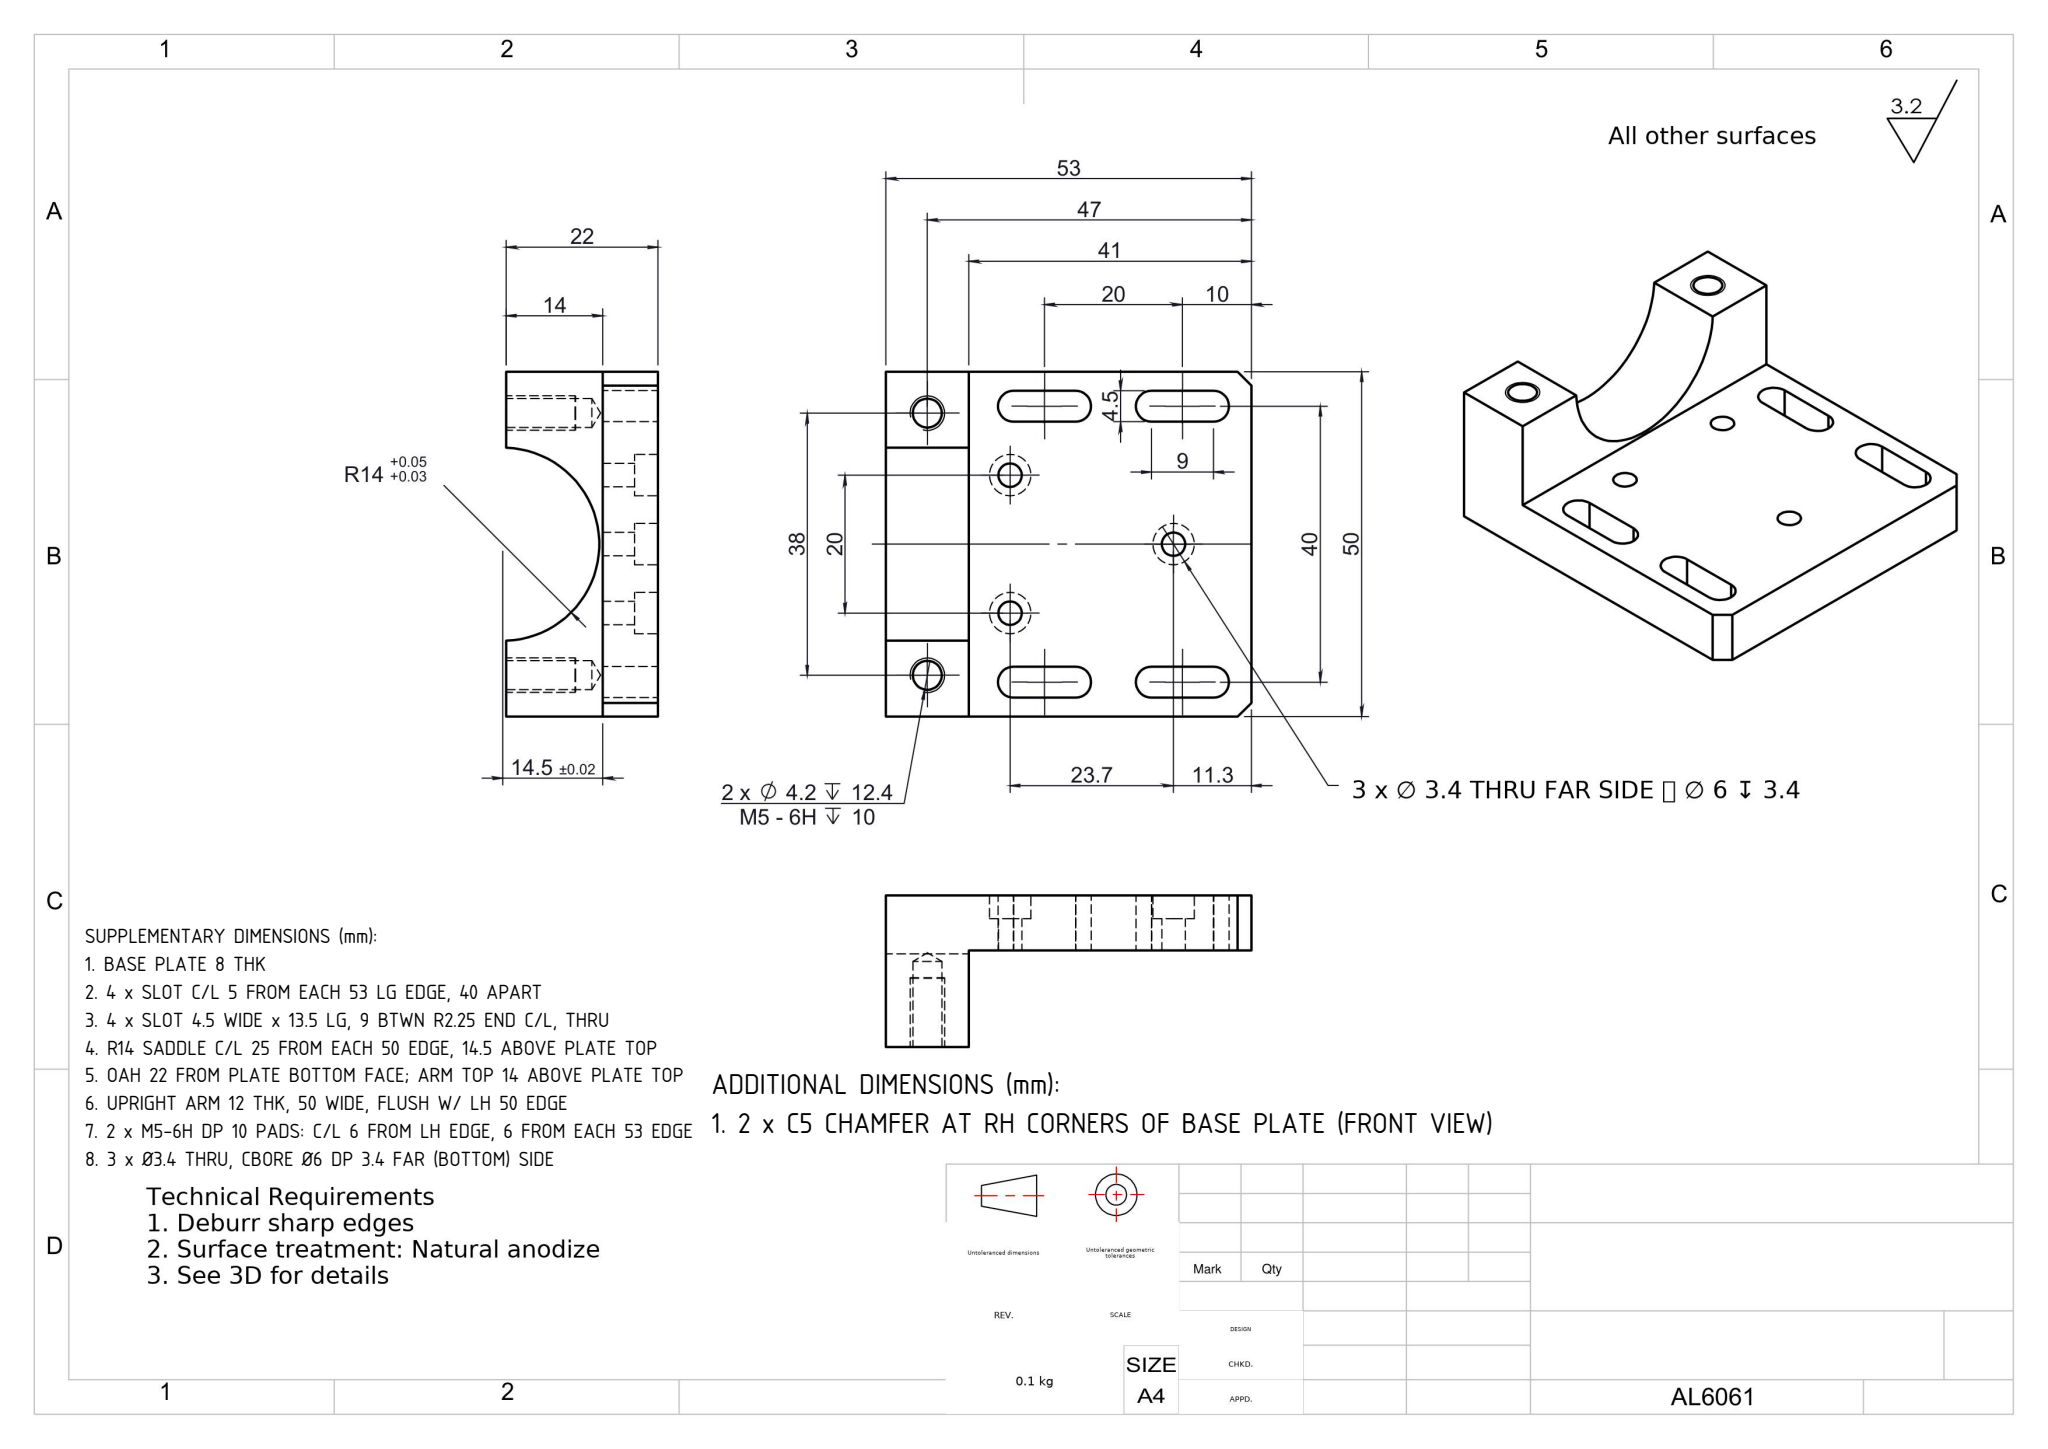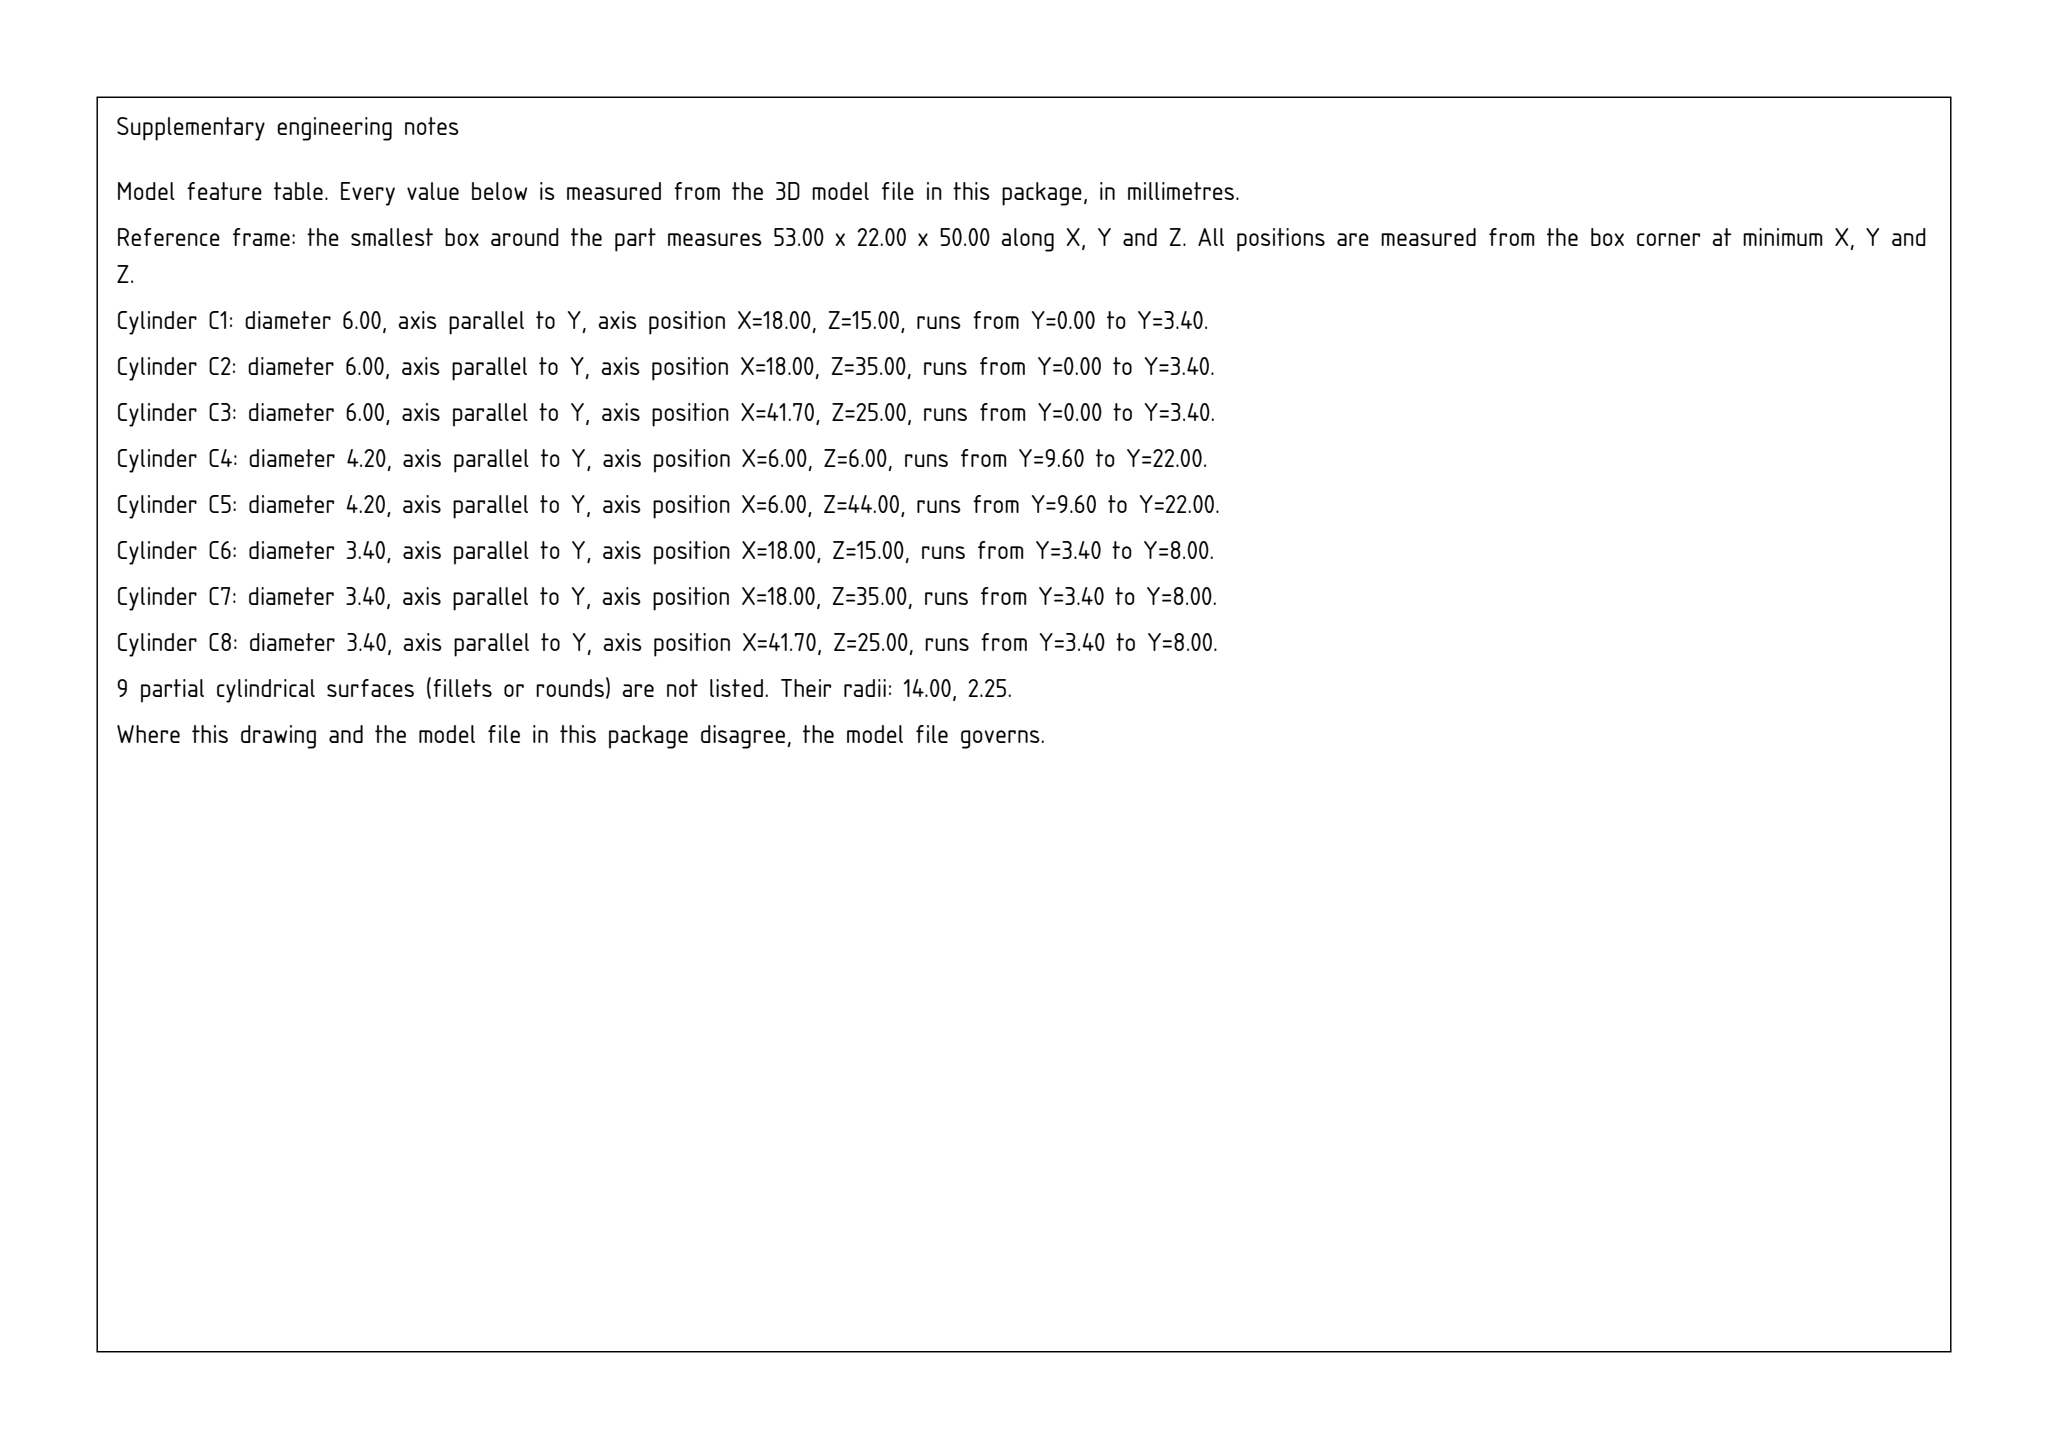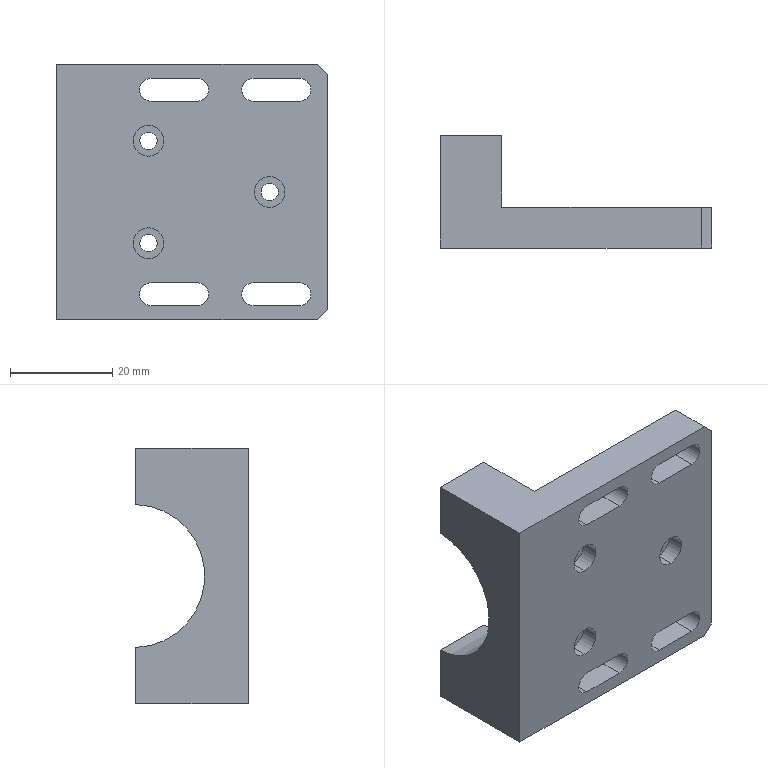Part | SolidWorks | mm | 1 solid | 51 faces | box 53 x 22 x 50 mm | volume 23468 mm3 | cylinder 25 | plane 22 | cone 4 | commonest cylinder face diameters 4.5 x8 6 x6 3.4 x6 4.2 x4 28 x1